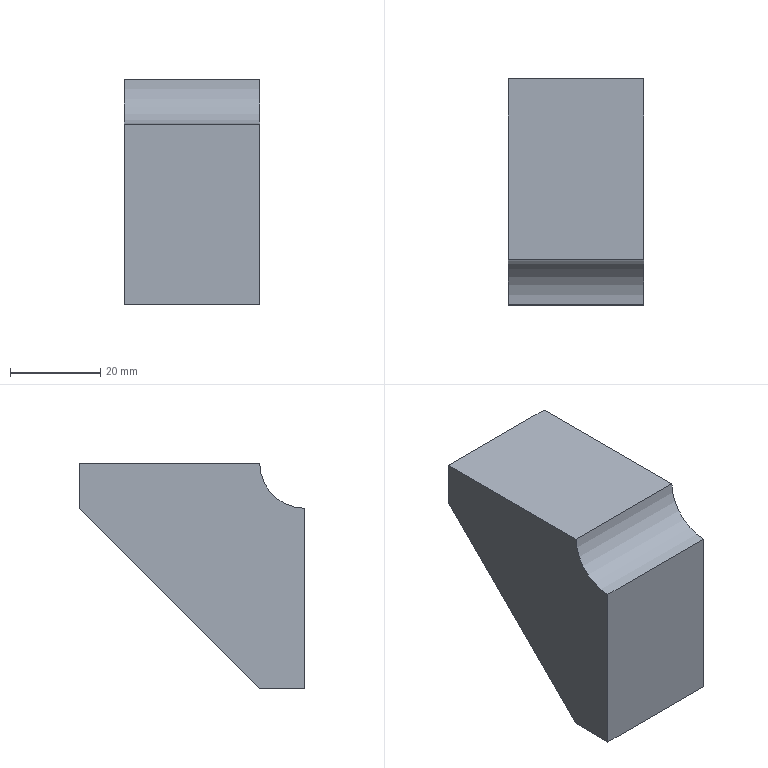Component | SolidWorks | JF21-80.1-1-3(_)-1-SOLID22-1 | 1 solid | 8 faces | box 30 x 50 x 50 mm | volume 48644 mm3 | plane 7 | cylinder 1 | commonest cylinder face diameters 20 x1
STEP:
#1=COLOUR_RGB('',0.7922,0.8196,0.9333);
#2=FILL_AREA_STYLE_COLOUR('',#1);
#3=FILL_AREA_STYLE('',(#2));
#4=SURFACE_STYLE_FILL_AREA(#3);
#5=SURFACE_SIDE_STYLE('',(#4));
#6=SURFACE_STYLE_USAGE(.BOTH.,#5);
#7=PRESENTATION_STYLE_ASSIGNMENT((#6));
#8=CARTESIAN_POINT('',(-0.5906,5.512,7.677));
#9=VERTEX_POINT('',#8);
#10=CARTESIAN_POINT('',(-0.5906,5.906,7.677));
#11=VERTEX_POINT('',#10);
#12=CARTESIAN_POINT('',(-0.5906,5.512,7.677));
#13=DIRECTION('',(0.,1.,0.));
#14=VECTOR('',#13,39.37);
#15=LINE('',#12,#14);
#16=EDGE_CURVE('',#9,#11,#15,.T.);
#17=ORIENTED_EDGE('',*,*,#16,.T.);
#18=CARTESIAN_POINT('',(0.5906,5.906,7.677));
#19=VERTEX_POINT('',#18);
#20=CARTESIAN_POINT('',(0.5906,5.906,7.677));
#21=DIRECTION('',(-1.,0.,0.));
#22=VECTOR('',#21,39.37);
#23=LINE('',#20,#22);
#24=EDGE_CURVE('',#19,#11,#23,.T.);
#25=ORIENTED_EDGE('',*,*,#24,.F.);
#26=CARTESIAN_POINT('',(0.5906,5.512,7.677));
#27=VERTEX_POINT('',#26);
#28=CARTESIAN_POINT('',(0.5906,5.512,7.677));
#29=DIRECTION('',(0.,1.,0.));
#30=VECTOR('',#29,39.37);
#31=LINE('',#28,#30);
#32=EDGE_CURVE('',#27,#19,#31,.T.);
#33=ORIENTED_EDGE('',*,*,#32,.F.);
#34=CARTESIAN_POINT('',(0.5906,5.512,7.677));
#35=DIRECTION('',(-1.,0.,0.));
#36=VECTOR('',#35,39.37);
#37=LINE('',#34,#36);
#38=EDGE_CURVE('',#27,#9,#37,.T.);
#39=ORIENTED_EDGE('',*,*,#38,.T.);
#40=EDGE_LOOP('',(#17,#25,#33,#39));
#41=FACE_OUTER_BOUND('',#40,.T.);
#42=CARTESIAN_POINT('',(0.5906,5.512,7.677));
#43=DIRECTION('',(0.,0.,1.));
#44=DIRECTION('',(-1.,0.,0.));
#45=AXIS2_PLACEMENT_3D('',#42,#43,#44);
#46=PLANE('',#45);
#47=ADVANCED_FACE('',(#41),#46,.F.);
#48=CARTESIAN_POINT('',(-0.5906,7.48,9.252));
#49=VERTEX_POINT('',#48);
#50=CARTESIAN_POINT('',(-0.5906,5.906,7.677));
#51=DIRECTION('',(0.,0.7071,0.7071));
#52=VECTOR('',#51,39.37);
#53=LINE('',#50,#52);
#54=EDGE_CURVE('',#11,#49,#53,.T.);
#55=ORIENTED_EDGE('',*,*,#54,.T.);
#56=CARTESIAN_POINT('',(0.5906,7.48,9.252));
#57=VERTEX_POINT('',#56);
#58=CARTESIAN_POINT('',(0.5906,7.48,9.252));
#59=DIRECTION('',(-1.,0.,0.));
#60=VECTOR('',#59,39.37);
#61=LINE('',#58,#60);
#62=EDGE_CURVE('',#57,#49,#61,.T.);
#63=ORIENTED_EDGE('',*,*,#62,.F.);
#64=CARTESIAN_POINT('',(0.5906,5.906,7.677));
#65=DIRECTION('',(0.,0.7071,0.7071));
#66=VECTOR('',#65,39.37);
#67=LINE('',#64,#66);
#68=EDGE_CURVE('',#19,#57,#67,.T.);
#69=ORIENTED_EDGE('',*,*,#68,.F.);
#70=ORIENTED_EDGE('',*,*,#24,.T.);
#71=EDGE_LOOP('',(#55,#63,#69,#70));
#72=FACE_OUTER_BOUND('',#71,.T.);
#73=CARTESIAN_POINT('',(0.5906,5.906,7.677));
#74=DIRECTION('',(0.,-0.7071,0.7071));
#75=DIRECTION('',(0.,0.7071,0.7071));
#76=AXIS2_PLACEMENT_3D('',#73,#74,#75);
#77=PLANE('',#76);
#78=ADVANCED_FACE('',(#72),#77,.F.);
#79=CARTESIAN_POINT('',(-0.5906,7.48,9.646));
#80=VERTEX_POINT('',#79);
#81=CARTESIAN_POINT('',(-0.5906,7.48,9.252));
#82=DIRECTION('',(0.,0.,1.));
#83=VECTOR('',#82,39.37);
#84=LINE('',#81,#83);
#85=EDGE_CURVE('',#49,#80,#84,.T.);
#86=ORIENTED_EDGE('',*,*,#85,.T.);
#87=CARTESIAN_POINT('',(0.5906,7.48,9.646));
#88=VERTEX_POINT('',#87);
#89=CARTESIAN_POINT('',(0.5906,7.48,9.646));
#90=DIRECTION('',(-1.,0.,0.));
#91=VECTOR('',#90,39.37);
#92=LINE('',#89,#91);
#93=EDGE_CURVE('',#88,#80,#92,.T.);
#94=ORIENTED_EDGE('',*,*,#93,.F.);
#95=CARTESIAN_POINT('',(0.5906,7.48,9.252));
#96=DIRECTION('',(0.,0.,1.));
#97=VECTOR('',#96,39.37);
#98=LINE('',#95,#97);
#99=EDGE_CURVE('',#57,#88,#98,.T.);
#100=ORIENTED_EDGE('',*,*,#99,.F.);
#101=ORIENTED_EDGE('',*,*,#62,.T.);
#102=EDGE_LOOP('',(#86,#94,#100,#101));
#103=FACE_OUTER_BOUND('',#102,.T.);
#104=CARTESIAN_POINT('',(0.5906,7.48,9.252));
#105=DIRECTION('',(0.,-1.,0.));
#106=DIRECTION('',(0.,0.,1.));
#107=AXIS2_PLACEMENT_3D('',#104,#105,#106);
#108=PLANE('',#107);
#109=ADVANCED_FACE('',(#103),#108,.F.);
#110=CARTESIAN_POINT('',(-0.5906,5.906,9.646));
#111=VERTEX_POINT('',#110);
#112=CARTESIAN_POINT('',(-0.5906,7.48,9.646));
#113=DIRECTION('',(0.,-1.,0.));
#114=VECTOR('',#113,39.37);
#115=LINE('',#112,#114);
#116=EDGE_CURVE('',#80,#111,#115,.T.);
#117=ORIENTED_EDGE('',*,*,#116,.T.);
#118=CARTESIAN_POINT('',(0.5906,5.906,9.646));
#119=VERTEX_POINT('',#118);
#120=CARTESIAN_POINT('',(0.5906,5.906,9.646));
#121=DIRECTION('',(-1.,0.,0.));
#122=VECTOR('',#121,39.37);
#123=LINE('',#120,#122);
#124=EDGE_CURVE('',#119,#111,#123,.T.);
#125=ORIENTED_EDGE('',*,*,#124,.F.);
#126=CARTESIAN_POINT('',(0.5906,7.48,9.646));
#127=DIRECTION('',(0.,-1.,0.));
#128=VECTOR('',#127,39.37);
#129=LINE('',#126,#128);
#130=EDGE_CURVE('',#88,#119,#129,.T.);
#131=ORIENTED_EDGE('',*,*,#130,.F.);
#132=ORIENTED_EDGE('',*,*,#93,.T.);
#133=EDGE_LOOP('',(#117,#125,#131,#132));
#134=FACE_OUTER_BOUND('',#133,.T.);
#135=CARTESIAN_POINT('',(0.5906,7.48,9.646));
#136=DIRECTION('',(0.,0.,-1.));
#137=DIRECTION('',(1.,0.,0.));
#138=AXIS2_PLACEMENT_3D('',#135,#136,#137);
#139=PLANE('',#138);
#140=ADVANCED_FACE('',(#134),#139,.F.);
#141=CARTESIAN_POINT('',(-0.5906,5.512,9.252));
#142=VERTEX_POINT('',#141);
#143=CARTESIAN_POINT('',(-0.5906,5.512,9.646));
#144=DIRECTION('',(-1.,0.,0.));
#145=DIRECTION('',(0.,0.,-1.));
#146=AXIS2_PLACEMENT_3D('',#143,#144,#145);
#147=CIRCLE('',#146,0.3937);
#148=EDGE_CURVE('',#111,#142,#147,.T.);
#149=ORIENTED_EDGE('',*,*,#148,.T.);
#150=CARTESIAN_POINT('',(0.5906,5.512,9.252));
#151=VERTEX_POINT('',#150);
#152=CARTESIAN_POINT('',(0.5906,5.512,9.252));
#153=DIRECTION('',(-1.,0.,0.));
#154=VECTOR('',#153,39.37);
#155=LINE('',#152,#154);
#156=EDGE_CURVE('',#151,#142,#155,.T.);
#157=ORIENTED_EDGE('',*,*,#156,.F.);
#158=CARTESIAN_POINT('',(0.5906,5.512,9.646));
#159=DIRECTION('',(-1.,0.,0.));
#160=DIRECTION('',(0.,0.,-1.));
#161=AXIS2_PLACEMENT_3D('',#158,#159,#160);
#162=CIRCLE('',#161,0.3937);
#163=EDGE_CURVE('',#119,#151,#162,.T.);
#164=ORIENTED_EDGE('',*,*,#163,.F.);
#165=ORIENTED_EDGE('',*,*,#124,.T.);
#166=EDGE_LOOP('',(#149,#157,#164,#165));
#167=FACE_OUTER_BOUND('',#166,.T.);
#168=CARTESIAN_POINT('',(0.5906,5.512,9.646));
#169=DIRECTION('',(-1.,0.,0.));
#170=DIRECTION('',(0.,0.,-1.));
#171=AXIS2_PLACEMENT_3D('',#168,#169,#170);
#172=CYLINDRICAL_SURFACE('',#171,0.3937);
#173=ADVANCED_FACE('',(#167),#172,.F.);
#174=CARTESIAN_POINT('',(-0.5906,5.512,9.252));
#175=DIRECTION('',(0.,0.,-1.));
#176=VECTOR('',#175,39.37);
#177=LINE('',#174,#176);
#178=EDGE_CURVE('',#142,#9,#177,.T.);
#179=ORIENTED_EDGE('',*,*,#178,.T.);
#180=ORIENTED_EDGE('',*,*,#38,.F.);
#181=CARTESIAN_POINT('',(0.5906,5.512,9.252));
#182=DIRECTION('',(0.,0.,-1.));
#183=VECTOR('',#182,39.37);
#184=LINE('',#181,#183);
#185=EDGE_CURVE('',#151,#27,#184,.T.);
#186=ORIENTED_EDGE('',*,*,#185,.F.);
#187=ORIENTED_EDGE('',*,*,#156,.T.);
#188=EDGE_LOOP('',(#179,#180,#186,#187));
#189=FACE_OUTER_BOUND('',#188,.T.);
#190=CARTESIAN_POINT('',(0.5906,5.512,9.252));
#191=DIRECTION('',(0.,1.,0.));
#192=DIRECTION('',(0.,0.,-1.));
#193=AXIS2_PLACEMENT_3D('',#190,#191,#192);
#194=PLANE('',#193);
#195=ADVANCED_FACE('',(#189),#194,.F.);
#196=ORIENTED_EDGE('',*,*,#32,.T.);
#197=ORIENTED_EDGE('',*,*,#68,.T.);
#198=ORIENTED_EDGE('',*,*,#99,.T.);
#199=ORIENTED_EDGE('',*,*,#130,.T.);
#200=ORIENTED_EDGE('',*,*,#163,.T.);
#201=ORIENTED_EDGE('',*,*,#185,.T.);
#202=EDGE_LOOP('',(#196,#197,#198,#199,#200,#201));
#203=FACE_OUTER_BOUND('',#202,.T.);
#204=CARTESIAN_POINT('',(0.5906,5.512,9.646));
#205=DIRECTION('',(1.,0.,0.));
#206=DIRECTION('',(0.,0.,1.));
#207=AXIS2_PLACEMENT_3D('',#204,#205,#206);
#208=PLANE('',#207);
#209=ADVANCED_FACE('',(#203),#208,.T.);
#210=ORIENTED_EDGE('',*,*,#16,.F.);
#211=ORIENTED_EDGE('',*,*,#178,.F.);
#212=ORIENTED_EDGE('',*,*,#148,.F.);
#213=ORIENTED_EDGE('',*,*,#116,.F.);
#214=ORIENTED_EDGE('',*,*,#85,.F.);
#215=ORIENTED_EDGE('',*,*,#54,.F.);
#216=EDGE_LOOP('',(#210,#211,#212,#213,#214,#215));
#217=FACE_OUTER_BOUND('',#216,.T.);
#218=CARTESIAN_POINT('',(-0.5906,5.512,9.646));
#219=DIRECTION('',(1.,0.,0.));
#220=DIRECTION('',(0.,0.,1.));
#221=AXIS2_PLACEMENT_3D('',#218,#219,#220);
#222=PLANE('',#221);
#223=ADVANCED_FACE('',(#217),#222,.F.);
#224=CLOSED_SHELL('',(#47,#78,#109,#140,#173,#195,#209,#223));
#225=MANIFOLD_SOLID_BREP('',#224);
#226=STYLED_ITEM('',(#7),#225);
#227=PRESENTATION_LAYER_ASSIGNMENT('','',(#226));
#228=(LENGTH_UNIT()NAMED_UNIT(*)SI_UNIT($,.METRE.));
#229=LENGTH_MEASURE_WITH_UNIT(LENGTH_MEASURE(0.0254),#228);
#230=DIMENSIONAL_EXPONENTS(1.,0.,0.,0.,0.,0.,0.);
#231=(CONVERSION_BASED_UNIT('',#229)LENGTH_UNIT()NAMED_UNIT(#230));
#232=UNCERTAINTY_MEASURE_WITH_UNIT(LENGTH_MEASURE(0.00001),#231,'','');
#233=(NAMED_UNIT(*)PLANE_ANGLE_UNIT()SI_UNIT($,.RADIAN.));
#234=(NAMED_UNIT(*)SI_UNIT($,.STERADIAN.)SOLID_ANGLE_UNIT());
#235=(GEOMETRIC_REPRESENTATION_CONTEXT(3)GLOBAL_UNCERTAINTY_ASSIGNED_CONTEXT((#232))GLOBAL_UNIT_ASSIGNED_CONTEXT((#231,#233,#234))REPRESENTATION_CONTEXT('',''));
#236=MECHANICAL_DESIGN_GEOMETRIC_PRESENTATION_REPRESENTATION('',(#226),#235);
#237=CARTESIAN_POINT('',(0.,0.,0.));
#238=DIRECTION('',(0.,0.,1.));
#239=DIRECTION('',(1.,0.,0.));
#240=AXIS2_PLACEMENT_3D('',#237,#238,#239);
#241=(LENGTH_UNIT()NAMED_UNIT(*)SI_UNIT($,.METRE.));
#242=LENGTH_MEASURE_WITH_UNIT(LENGTH_MEASURE(0.0254),#241);
#243=DIMENSIONAL_EXPONENTS(1.,0.,0.,0.,0.,0.,0.);
#244=(CONVERSION_BASED_UNIT('',#242)LENGTH_UNIT()NAMED_UNIT(#243));
#245=UNCERTAINTY_MEASURE_WITH_UNIT(LENGTH_MEASURE(0.00001),#244,'','');
#246=(NAMED_UNIT(*)PLANE_ANGLE_UNIT()SI_UNIT($,.RADIAN.));
#247=(NAMED_UNIT(*)SI_UNIT($,.STERADIAN.)SOLID_ANGLE_UNIT());
#248=(GEOMETRIC_REPRESENTATION_CONTEXT(3)GLOBAL_UNCERTAINTY_ASSIGNED_CONTEXT((#245))GLOBAL_UNIT_ASSIGNED_CONTEXT((#244,#246,#247))REPRESENTATION_CONTEXT('',''));
#249=ADVANCED_BREP_SHAPE_REPRESENTATION('',(#225,#240),#248);